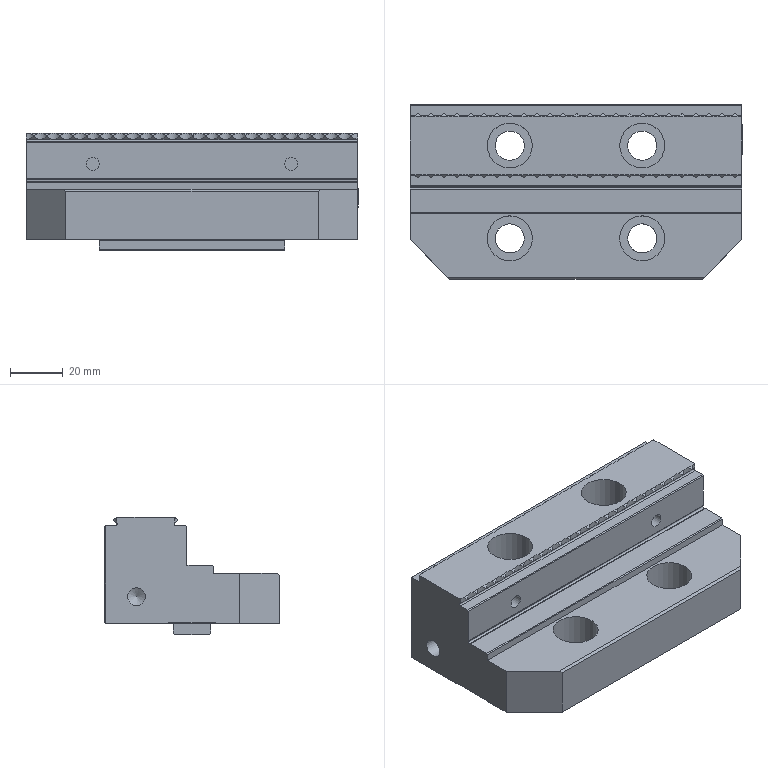Component | NX | JAW_MOVING_125 | 1 solid | 281 faces | volume 216184 mm3 | plane 195 | cylinder 81 | cone 5 | commonest cylinder face diameters 6 x52 11 x4 17 x4 13 x4 2 x4 1 x3 6.65 x3 6.8 x2